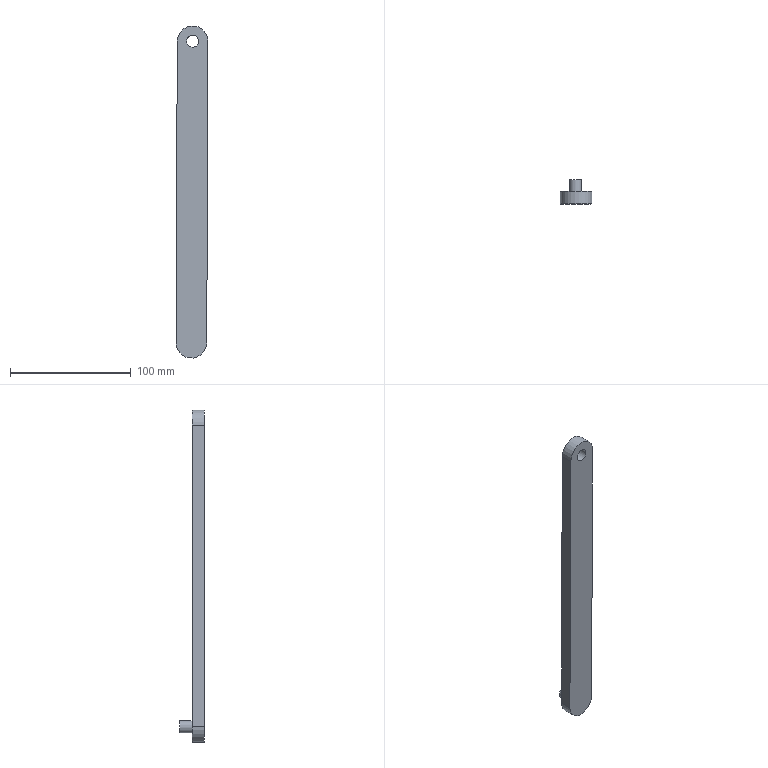Component | NX | 07 | 1 solid | 9 faces | box 26.54 x 20 x 275.49 mm | volume 68832 mm3 | plane 5 | cylinder 4 | commonest cylinder face diameters 25.491 x2 10 x2
STEP:
#1=CARTESIAN_POINT('',(0.,0.,0.));
#2=DIRECTION('',(0.,0.,1.));
#3=DIRECTION('',(1.,0.,0.));
#4=AXIS2_PLACEMENT_3D('',#1,#2,#3);
#5=CARTESIAN_POINT('',(-187.255,5.,90.359));
#6=VERTEX_POINT('',#5);
#7=CARTESIAN_POINT('',(-186.21,5.,340.356));
#8=VERTEX_POINT('',#7);
#9=CARTESIAN_POINT('',(-187.255,5.,90.359));
#10=DIRECTION('',(0.004176,0.,1.));
#11=VECTOR('',#10,1.);
#12=LINE('',#9,#11);
#13=CARTESIAN_POINT('',(-187.255,15.,90.359));
#14=DIRECTION('',(1.,0.,-0.004176));
#15=DIRECTION('',(-0.004176,0.,-1.));
#16=AXIS2_PLACEMENT_3D('',#13,#14,#15);
#17=PLANE('',#16);
#18=CARTESIAN_POINT('',(0.,-10.));
#19=DIRECTION('',(-1.,0.));
#20=VECTOR('',#19,1.);
#21=LINE('',#18,#20);
#22=(GEOMETRIC_REPRESENTATION_CONTEXT(2)PARAMETRIC_REPRESENTATION_CONTEXT()REPRESENTATION_CONTEXT('',''));
#23=DEFINITIONAL_REPRESENTATION('',(#21),#22);
#24=PCURVE('',#17,#23);
#25=CARTESIAN_POINT('',(-198.956,5.,340.41));
#26=DIRECTION('',(0.,-1.,0.));
#27=DIRECTION('',(0.004176,0.,1.));
#28=AXIS2_PLACEMENT_3D('',#25,#26,#27);
#29=PLANE('',#28);
#30=CARTESIAN_POINT('',(-250.,-12.746));
#31=DIRECTION('',(1.,0.));
#32=VECTOR('',#31,1.);
#33=LINE('',#30,#32);
#34=(GEOMETRIC_REPRESENTATION_CONTEXT(2)PARAMETRIC_REPRESENTATION_CONTEXT()REPRESENTATION_CONTEXT('',''));
#35=DEFINITIONAL_REPRESENTATION('',(#33),#34);
#36=PCURVE('',#29,#35);
#37=SURFACE_CURVE('',#12,(#24,#36),.PCURVE_S1.);
#38=EDGE_CURVE('',#6,#8,#37,.T.);
#39=ORIENTED_EDGE('',*,*,#38,.F.);
#40=CARTESIAN_POINT('',(-187.255,15.,90.359));
#41=VERTEX_POINT('',#40);
#42=CARTESIAN_POINT('',(-187.255,15.,90.359));
#43=DIRECTION('',(0.,-1.,0.));
#44=VECTOR('',#43,1.);
#45=LINE('',#42,#44);
#46=CARTESIAN_POINT('',(0.,0.));
#47=DIRECTION('',(0.,-1.));
#48=VECTOR('',#47,1.);
#49=LINE('',#46,#48);
#50=(GEOMETRIC_REPRESENTATION_CONTEXT(2)PARAMETRIC_REPRESENTATION_CONTEXT()REPRESENTATION_CONTEXT('',''));
#51=DEFINITIONAL_REPRESENTATION('',(#49),#50);
#52=PCURVE('',#17,#51);
#53=CARTESIAN_POINT('',(-200.,15.,90.412));
#54=DIRECTION('',(0.,-1.,0.));
#55=DIRECTION('',(0.004176,0.,1.));
#56=AXIS2_PLACEMENT_3D('',#53,#54,#55);
#57=CYLINDRICAL_SURFACE('',#56,12.746);
#58=CARTESIAN_POINT('',(4.712,0.));
#59=DIRECTION('',(0.,1.));
#60=VECTOR('',#59,1.);
#61=LINE('',#58,#60);
#62=(GEOMETRIC_REPRESENTATION_CONTEXT(2)PARAMETRIC_REPRESENTATION_CONTEXT()REPRESENTATION_CONTEXT('',''));
#63=DEFINITIONAL_REPRESENTATION('',(#61),#62);
#64=PCURVE('',#57,#63);
#65=SURFACE_CURVE('',#45,(#52,#64),.PCURVE_S1.);
#66=EDGE_CURVE('',#41,#6,#65,.T.);
#67=ORIENTED_EDGE('',*,*,#66,.F.);
#68=CARTESIAN_POINT('',(-186.21,15.,340.356));
#69=VERTEX_POINT('',#68);
#70=CARTESIAN_POINT('',(-187.255,15.,90.359));
#71=DIRECTION('',(0.004176,0.,1.));
#72=VECTOR('',#71,1.);
#73=LINE('',#70,#72);
#74=CARTESIAN_POINT('',(0.,0.));
#75=DIRECTION('',(-1.,0.));
#76=VECTOR('',#75,1.);
#77=LINE('',#74,#76);
#78=(GEOMETRIC_REPRESENTATION_CONTEXT(2)PARAMETRIC_REPRESENTATION_CONTEXT()REPRESENTATION_CONTEXT('',''));
#79=DEFINITIONAL_REPRESENTATION('',(#77),#78);
#80=PCURVE('',#17,#79);
#81=CARTESIAN_POINT('',(-198.956,15.,340.41));
#82=DIRECTION('',(0.,-1.,0.));
#83=DIRECTION('',(0.004176,0.,1.));
#84=AXIS2_PLACEMENT_3D('',#81,#82,#83);
#85=PLANE('',#84);
#86=CARTESIAN_POINT('',(-250.,-12.746));
#87=DIRECTION('',(1.,0.));
#88=VECTOR('',#87,1.);
#89=LINE('',#86,#88);
#90=(GEOMETRIC_REPRESENTATION_CONTEXT(2)PARAMETRIC_REPRESENTATION_CONTEXT()REPRESENTATION_CONTEXT('',''));
#91=DEFINITIONAL_REPRESENTATION('',(#89),#90);
#92=PCURVE('',#85,#91);
#93=SURFACE_CURVE('',#73,(#80,#92),.PCURVE_S1.);
#94=EDGE_CURVE('',#41,#69,#93,.T.);
#95=ORIENTED_EDGE('',*,*,#94,.T.);
#96=CARTESIAN_POINT('',(-186.21,15.,340.356));
#97=DIRECTION('',(0.,-1.,0.));
#98=VECTOR('',#97,1.);
#99=LINE('',#96,#98);
#100=CARTESIAN_POINT('',(-250.,0.));
#101=DIRECTION('',(0.,-1.));
#102=VECTOR('',#101,1.);
#103=LINE('',#100,#102);
#104=(GEOMETRIC_REPRESENTATION_CONTEXT(2)PARAMETRIC_REPRESENTATION_CONTEXT()REPRESENTATION_CONTEXT('',''));
#105=DEFINITIONAL_REPRESENTATION('',(#103),#104);
#106=PCURVE('',#17,#105);
#107=CARTESIAN_POINT('',(-198.956,15.,340.41));
#108=DIRECTION('',(0.,-1.,0.));
#109=DIRECTION('',(0.004176,0.,1.));
#110=AXIS2_PLACEMENT_3D('',#107,#108,#109);
#111=CYLINDRICAL_SURFACE('',#110,12.746);
#112=CARTESIAN_POINT('',(-1.571,0.));
#113=DIRECTION('',(0.,1.));
#114=VECTOR('',#113,1.);
#115=LINE('',#112,#114);
#116=(GEOMETRIC_REPRESENTATION_CONTEXT(2)PARAMETRIC_REPRESENTATION_CONTEXT()REPRESENTATION_CONTEXT('',''));
#117=DEFINITIONAL_REPRESENTATION('',(#115),#116);
#118=PCURVE('',#111,#117);
#119=SURFACE_CURVE('',#99,(#106,#118),.PCURVE_S1.);
#120=EDGE_CURVE('',#69,#8,#119,.T.);
#121=ORIENTED_EDGE('',*,*,#120,.T.);
#122=EDGE_LOOP('',(#39,#67,#95,#121));
#123=FACE_BOUND('',#122,.T.);
#124=ADVANCED_FACE('',(#123),#17,.T.);
#125=CARTESIAN_POINT('',(-211.701,5.,340.463));
#126=VERTEX_POINT('',#125);
#127=CARTESIAN_POINT('',(-198.956,5.,340.41));
#128=DIRECTION('',(0.,-1.,0.));
#129=DIRECTION('',(-1.,0.,0.004176));
#130=AXIS2_PLACEMENT_3D('',#127,#128,#129);
#131=CIRCLE('',#130,12.746);
#132=CARTESIAN_POINT('',(-4.712,10.));
#133=DIRECTION('',(1.,0.));
#134=VECTOR('',#133,1.);
#135=LINE('',#132,#134);
#136=(GEOMETRIC_REPRESENTATION_CONTEXT(2)PARAMETRIC_REPRESENTATION_CONTEXT()REPRESENTATION_CONTEXT('',''));
#137=DEFINITIONAL_REPRESENTATION('',(#135),#136);
#138=PCURVE('',#111,#137);
#139=CARTESIAN_POINT('',(0.,0.));
#140=DIRECTION('',(0.,1.));
#141=AXIS2_PLACEMENT_2D('',#139,#140);
#142=CIRCLE('',#141,12.746);
#143=(GEOMETRIC_REPRESENTATION_CONTEXT(2)PARAMETRIC_REPRESENTATION_CONTEXT()REPRESENTATION_CONTEXT('',''));
#144=DEFINITIONAL_REPRESENTATION('',(#142),#143);
#145=PCURVE('',#29,#144);
#146=SURFACE_CURVE('',#131,(#138,#145),.PCURVE_S1.);
#147=EDGE_CURVE('',#8,#126,#146,.T.);
#148=ORIENTED_EDGE('',*,*,#147,.F.);
#149=ORIENTED_EDGE('',*,*,#120,.F.);
#150=CARTESIAN_POINT('',(-211.701,15.,340.463));
#151=VERTEX_POINT('',#150);
#152=CARTESIAN_POINT('',(-198.956,15.,340.41));
#153=DIRECTION('',(0.,-1.,0.));
#154=DIRECTION('',(-1.,0.,0.004176));
#155=AXIS2_PLACEMENT_3D('',#152,#153,#154);
#156=CIRCLE('',#155,12.746);
#157=CARTESIAN_POINT('',(-4.712,0.));
#158=DIRECTION('',(1.,0.));
#159=VECTOR('',#158,1.);
#160=LINE('',#157,#159);
#161=(GEOMETRIC_REPRESENTATION_CONTEXT(2)PARAMETRIC_REPRESENTATION_CONTEXT()REPRESENTATION_CONTEXT('',''));
#162=DEFINITIONAL_REPRESENTATION('',(#160),#161);
#163=PCURVE('',#111,#162);
#164=CARTESIAN_POINT('',(0.,0.));
#165=DIRECTION('',(0.,1.));
#166=AXIS2_PLACEMENT_2D('',#164,#165);
#167=CIRCLE('',#166,12.746);
#168=(GEOMETRIC_REPRESENTATION_CONTEXT(2)PARAMETRIC_REPRESENTATION_CONTEXT()REPRESENTATION_CONTEXT('',''));
#169=DEFINITIONAL_REPRESENTATION('',(#167),#168);
#170=PCURVE('',#85,#169);
#171=SURFACE_CURVE('',#156,(#163,#170),.PCURVE_S1.);
#172=EDGE_CURVE('',#69,#151,#171,.T.);
#173=ORIENTED_EDGE('',*,*,#172,.T.);
#174=CARTESIAN_POINT('',(-211.701,15.,340.463));
#175=DIRECTION('',(0.,-1.,0.));
#176=VECTOR('',#175,1.);
#177=LINE('',#174,#176);
#178=CARTESIAN_POINT('',(1.571,0.));
#179=DIRECTION('',(0.,1.));
#180=VECTOR('',#179,1.);
#181=LINE('',#178,#180);
#182=(GEOMETRIC_REPRESENTATION_CONTEXT(2)PARAMETRIC_REPRESENTATION_CONTEXT()REPRESENTATION_CONTEXT('',''));
#183=DEFINITIONAL_REPRESENTATION('',(#181),#182);
#184=PCURVE('',#111,#183);
#185=CARTESIAN_POINT('',(-211.701,15.,340.463));
#186=DIRECTION('',(-1.,0.,0.004176));
#187=DIRECTION('',(0.004176,0.,1.));
#188=AXIS2_PLACEMENT_3D('',#185,#186,#187);
#189=PLANE('',#188);
#190=CARTESIAN_POINT('',(0.,0.));
#191=DIRECTION('',(0.,-1.));
#192=VECTOR('',#191,1.);
#193=LINE('',#190,#192);
#194=(GEOMETRIC_REPRESENTATION_CONTEXT(2)PARAMETRIC_REPRESENTATION_CONTEXT()REPRESENTATION_CONTEXT('',''));
#195=DEFINITIONAL_REPRESENTATION('',(#193),#194);
#196=PCURVE('',#189,#195);
#197=SURFACE_CURVE('',#177,(#184,#196),.PCURVE_S1.);
#198=EDGE_CURVE('',#151,#126,#197,.T.);
#199=ORIENTED_EDGE('',*,*,#198,.T.);
#200=EDGE_LOOP('',(#148,#149,#173,#199));
#201=FACE_BOUND('',#200,.T.);
#202=ADVANCED_FACE('',(#201),#111,.T.);
#203=CARTESIAN_POINT('',(-212.745,5.,90.465));
#204=VERTEX_POINT('',#203);
#205=CARTESIAN_POINT('',(-211.701,5.,340.463));
#206=DIRECTION('',(-0.004176,0.,-1.));
#207=VECTOR('',#206,1.);
#208=LINE('',#205,#207);
#209=CARTESIAN_POINT('',(0.,-10.));
#210=DIRECTION('',(-1.,0.));
#211=VECTOR('',#210,1.);
#212=LINE('',#209,#211);
#213=(GEOMETRIC_REPRESENTATION_CONTEXT(2)PARAMETRIC_REPRESENTATION_CONTEXT()REPRESENTATION_CONTEXT('',''));
#214=DEFINITIONAL_REPRESENTATION('',(#212),#213);
#215=PCURVE('',#189,#214);
#216=CARTESIAN_POINT('',(-0.,12.746));
#217=DIRECTION('',(-1.,-0.));
#218=VECTOR('',#217,1.);
#219=LINE('',#216,#218);
#220=(GEOMETRIC_REPRESENTATION_CONTEXT(2)PARAMETRIC_REPRESENTATION_CONTEXT()REPRESENTATION_CONTEXT('',''));
#221=DEFINITIONAL_REPRESENTATION('',(#219),#220);
#222=PCURVE('',#29,#221);
#223=SURFACE_CURVE('',#208,(#215,#222),.PCURVE_S1.);
#224=EDGE_CURVE('',#126,#204,#223,.T.);
#225=ORIENTED_EDGE('',*,*,#224,.F.);
#226=ORIENTED_EDGE('',*,*,#198,.F.);
#227=CARTESIAN_POINT('',(-212.745,15.,90.465));
#228=VERTEX_POINT('',#227);
#229=CARTESIAN_POINT('',(-211.701,15.,340.463));
#230=DIRECTION('',(-0.004176,0.,-1.));
#231=VECTOR('',#230,1.);
#232=LINE('',#229,#231);
#233=CARTESIAN_POINT('',(0.,0.));
#234=DIRECTION('',(-1.,0.));
#235=VECTOR('',#234,1.);
#236=LINE('',#233,#235);
#237=(GEOMETRIC_REPRESENTATION_CONTEXT(2)PARAMETRIC_REPRESENTATION_CONTEXT()REPRESENTATION_CONTEXT('',''));
#238=DEFINITIONAL_REPRESENTATION('',(#236),#237);
#239=PCURVE('',#189,#238);
#240=CARTESIAN_POINT('',(-0.,12.746));
#241=DIRECTION('',(-1.,-0.));
#242=VECTOR('',#241,1.);
#243=LINE('',#240,#242);
#244=(GEOMETRIC_REPRESENTATION_CONTEXT(2)PARAMETRIC_REPRESENTATION_CONTEXT()REPRESENTATION_CONTEXT('',''));
#245=DEFINITIONAL_REPRESENTATION('',(#243),#244);
#246=PCURVE('',#85,#245);
#247=SURFACE_CURVE('',#232,(#239,#246),.PCURVE_S1.);
#248=EDGE_CURVE('',#151,#228,#247,.T.);
#249=ORIENTED_EDGE('',*,*,#248,.T.);
#250=CARTESIAN_POINT('',(-212.745,15.,90.465));
#251=DIRECTION('',(0.,-1.,0.));
#252=VECTOR('',#251,1.);
#253=LINE('',#250,#252);
#254=CARTESIAN_POINT('',(-250.,0.));
#255=DIRECTION('',(0.,-1.));
#256=VECTOR('',#255,1.);
#257=LINE('',#254,#256);
#258=(GEOMETRIC_REPRESENTATION_CONTEXT(2)PARAMETRIC_REPRESENTATION_CONTEXT()REPRESENTATION_CONTEXT('',''));
#259=DEFINITIONAL_REPRESENTATION('',(#257),#258);
#260=PCURVE('',#189,#259);
#261=CARTESIAN_POINT('',(1.571,0.));
#262=DIRECTION('',(0.,1.));
#263=VECTOR('',#262,1.);
#264=LINE('',#261,#263);
#265=(GEOMETRIC_REPRESENTATION_CONTEXT(2)PARAMETRIC_REPRESENTATION_CONTEXT()REPRESENTATION_CONTEXT('',''));
#266=DEFINITIONAL_REPRESENTATION('',(#264),#265);
#267=PCURVE('',#57,#266);
#268=SURFACE_CURVE('',#253,(#260,#267),.PCURVE_S1.);
#269=EDGE_CURVE('',#228,#204,#268,.T.);
#270=ORIENTED_EDGE('',*,*,#269,.T.);
#271=EDGE_LOOP('',(#225,#226,#249,#270));
#272=FACE_BOUND('',#271,.T.);
#273=ADVANCED_FACE('',(#272),#189,.T.);
#274=CARTESIAN_POINT('',(-200.,5.,90.412));
#275=DIRECTION('',(0.,-1.,0.));
#276=DIRECTION('',(-1.,0.,0.004176));
#277=AXIS2_PLACEMENT_3D('',#274,#275,#276);
#278=CIRCLE('',#277,12.746);
#279=CARTESIAN_POINT('',(1.571,10.));
#280=DIRECTION('',(1.,0.));
#281=VECTOR('',#280,1.);
#282=LINE('',#279,#281);
#283=(GEOMETRIC_REPRESENTATION_CONTEXT(2)PARAMETRIC_REPRESENTATION_CONTEXT()REPRESENTATION_CONTEXT('',''));
#284=DEFINITIONAL_REPRESENTATION('',(#282),#283);
#285=PCURVE('',#57,#284);
#286=CARTESIAN_POINT('',(-250.,0.));
#287=DIRECTION('',(0.,1.));
#288=AXIS2_PLACEMENT_2D('',#286,#287);
#289=CIRCLE('',#288,12.746);
#290=(GEOMETRIC_REPRESENTATION_CONTEXT(2)PARAMETRIC_REPRESENTATION_CONTEXT()REPRESENTATION_CONTEXT('',''));
#291=DEFINITIONAL_REPRESENTATION('',(#289),#290);
#292=PCURVE('',#29,#291);
#293=SURFACE_CURVE('',#278,(#285,#292),.PCURVE_S1.);
#294=EDGE_CURVE('',#204,#6,#293,.T.);
#295=ORIENTED_EDGE('',*,*,#294,.F.);
#296=ORIENTED_EDGE('',*,*,#269,.F.);
#297=CARTESIAN_POINT('',(-200.,15.,90.412));
#298=DIRECTION('',(0.,-1.,0.));
#299=DIRECTION('',(-1.,0.,0.004176));
#300=AXIS2_PLACEMENT_3D('',#297,#298,#299);
#301=CIRCLE('',#300,12.746);
#302=CARTESIAN_POINT('',(1.571,0.));
#303=DIRECTION('',(1.,0.));
#304=VECTOR('',#303,1.);
#305=LINE('',#302,#304);
#306=(GEOMETRIC_REPRESENTATION_CONTEXT(2)PARAMETRIC_REPRESENTATION_CONTEXT()REPRESENTATION_CONTEXT('',''));
#307=DEFINITIONAL_REPRESENTATION('',(#305),#306);
#308=PCURVE('',#57,#307);
#309=CARTESIAN_POINT('',(-250.,0.));
#310=DIRECTION('',(0.,1.));
#311=AXIS2_PLACEMENT_2D('',#309,#310);
#312=CIRCLE('',#311,12.746);
#313=(GEOMETRIC_REPRESENTATION_CONTEXT(2)PARAMETRIC_REPRESENTATION_CONTEXT()REPRESENTATION_CONTEXT('',''));
#314=DEFINITIONAL_REPRESENTATION('',(#312),#313);
#315=PCURVE('',#85,#314);
#316=SURFACE_CURVE('',#301,(#308,#315),.PCURVE_S1.);
#317=EDGE_CURVE('',#228,#41,#316,.T.);
#318=ORIENTED_EDGE('',*,*,#317,.T.);
#319=ORIENTED_EDGE('',*,*,#66,.T.);
#320=EDGE_LOOP('',(#295,#296,#318,#319));
#321=FACE_BOUND('',#320,.T.);
#322=ADVANCED_FACE('',(#321),#57,.T.);
#323=CARTESIAN_POINT('',(-205.,15.,90.433));
#324=VERTEX_POINT('',#323);
#325=CARTESIAN_POINT('',(-200.,15.,90.412));
#326=DIRECTION('',(0.,1.,0.));
#327=DIRECTION('',(-1.,0.,0.004176));
#328=AXIS2_PLACEMENT_3D('',#325,#326,#327);
#329=CIRCLE('',#328,5.);
#330=CARTESIAN_POINT('',(-250.,5.));
#331=CARTESIAN_POINT('',(-241.34,5.));
#332=CARTESIAN_POINT('',(-245.67,-2.5));
#333=CARTESIAN_POINT('',(-250.,-10.));
#334=CARTESIAN_POINT('',(-254.33,-2.5));
#335=CARTESIAN_POINT('',(-258.66,5.));
#336=CARTESIAN_POINT('',(-250.,5.));
#337=(BOUNDED_CURVE()B_SPLINE_CURVE(2,(#330,#331,#332,#333,#334,#335,#336),.UNSPECIFIED.,.T.,.F.)B_SPLINE_CURVE_WITH_KNOTS((1,2,2,2,2,1),(-2.094,0.,2.094,4.189,6.283,8.378),.UNSPECIFIED.)CURVE()GEOMETRIC_REPRESENTATION_ITEM()RATIONAL_B_SPLINE_CURVE((1.,0.5,1.,0.5,1.,0.5,1.))REPRESENTATION_ITEM(''));
#338=(GEOMETRIC_REPRESENTATION_CONTEXT(2)PARAMETRIC_REPRESENTATION_CONTEXT()REPRESENTATION_CONTEXT('',''));
#339=DEFINITIONAL_REPRESENTATION('',(#337),#338);
#340=PCURVE('',#85,#339);
#341=CARTESIAN_POINT('',(-200.,25.,90.412));
#342=DIRECTION('',(0.,-1.,0.));
#343=DIRECTION('',(0.004176,0.,1.));
#344=AXIS2_PLACEMENT_3D('',#341,#342,#343);
#345=CYLINDRICAL_SURFACE('',#344,5.);
#346=CARTESIAN_POINT('',(7.854,10.));
#347=DIRECTION('',(-1.,0.));
#348=VECTOR('',#347,1.);
#349=LINE('',#346,#348);
#350=(GEOMETRIC_REPRESENTATION_CONTEXT(2)PARAMETRIC_REPRESENTATION_CONTEXT()REPRESENTATION_CONTEXT('',''));
#351=DEFINITIONAL_REPRESENTATION('',(#349),#350);
#352=PCURVE('',#345,#351);
#353=SURFACE_CURVE('',#329,(#340,#352),.PCURVE_S1.);
#354=EDGE_CURVE('',#324,#324,#353,.T.);
#355=ORIENTED_EDGE('',*,*,#354,.F.);
#356=EDGE_LOOP('',(#355));
#357=FACE_BOUND('',#356,.T.);
#358=CARTESIAN_POINT('',(-203.956,15.,340.431));
#359=VERTEX_POINT('',#358);
#360=CARTESIAN_POINT('',(-198.956,15.,340.41));
#361=DIRECTION('',(0.,1.,0.));
#362=DIRECTION('',(-1.,0.,0.004176));
#363=AXIS2_PLACEMENT_3D('',#360,#361,#362);
#364=CIRCLE('',#363,5.);
#365=CARTESIAN_POINT('',(0.,5.));
#366=CARTESIAN_POINT('',(8.66,5.));
#367=CARTESIAN_POINT('',(4.33,-2.5));
#368=CARTESIAN_POINT('',(-0.,-10.));
#369=CARTESIAN_POINT('',(-4.33,-2.5));
#370=CARTESIAN_POINT('',(-8.66,5.));
#371=CARTESIAN_POINT('',(0.,5.));
#372=(BOUNDED_CURVE()B_SPLINE_CURVE(2,(#365,#366,#367,#368,#369,#370,#371),.UNSPECIFIED.,.T.,.F.)B_SPLINE_CURVE_WITH_KNOTS((1,2,2,2,2,1),(-2.094,0.,2.094,4.189,6.283,8.378),.UNSPECIFIED.)CURVE()GEOMETRIC_REPRESENTATION_ITEM()RATIONAL_B_SPLINE_CURVE((1.,0.5,1.,0.5,1.,0.5,1.))REPRESENTATION_ITEM(''));
#373=(GEOMETRIC_REPRESENTATION_CONTEXT(2)PARAMETRIC_REPRESENTATION_CONTEXT()REPRESENTATION_CONTEXT('',''));
#374=DEFINITIONAL_REPRESENTATION('',(#372),#373);
#375=PCURVE('',#85,#374);
#376=CARTESIAN_POINT('',(-198.956,-84.,340.41));
#377=DIRECTION('',(0.,1.,0.));
#378=DIRECTION('',(-0.004176,0.,-1.));
#379=AXIS2_PLACEMENT_3D('',#376,#377,#378);
#380=CYLINDRICAL_SURFACE('',#379,5.);
#381=CARTESIAN_POINT('',(1.571,99.));
#382=DIRECTION('',(1.,0.));
#383=VECTOR('',#382,1.);
#384=LINE('',#381,#383);
#385=(GEOMETRIC_REPRESENTATION_CONTEXT(2)PARAMETRIC_REPRESENTATION_CONTEXT()REPRESENTATION_CONTEXT('',''));
#386=DEFINITIONAL_REPRESENTATION('',(#384),#385);
#387=PCURVE('',#380,#386);
#388=SURFACE_CURVE('',#364,(#375,#387),.PCURVE_S1.);
#389=EDGE_CURVE('',#359,#359,#388,.T.);
#390=ORIENTED_EDGE('',*,*,#389,.F.);
#391=EDGE_LOOP('',(#390));
#392=FACE_BOUND('',#391,.T.);
#393=ORIENTED_EDGE('',*,*,#94,.F.);
#394=ORIENTED_EDGE('',*,*,#317,.F.);
#395=ORIENTED_EDGE('',*,*,#248,.F.);
#396=ORIENTED_EDGE('',*,*,#172,.F.);
#397=EDGE_LOOP('',(#393,#394,#395,#396));
#398=FACE_BOUND('',#397,.T.);
#399=ADVANCED_FACE('',(#357,#392,#398),#85,.F.);
#400=CARTESIAN_POINT('',(-198.935,5.,345.41));
#401=VERTEX_POINT('',#400);
#402=CARTESIAN_POINT('',(-203.956,5.,340.431));
#403=VERTEX_POINT('',#402);
#404=CARTESIAN_POINT('',(-198.956,5.,340.41));
#405=DIRECTION('',(0.,1.,0.));
#406=DIRECTION('',(0.004176,0.,1.));
#407=AXIS2_PLACEMENT_3D('',#404,#405,#406);
#408=CIRCLE('',#407,5.);
#409=CARTESIAN_POINT('',(5.,0.));
#410=CARTESIAN_POINT('',(5.,-8.66));
#411=CARTESIAN_POINT('',(-2.5,-4.33));
#412=CARTESIAN_POINT('',(-10.,-0.));
#413=CARTESIAN_POINT('',(-2.5,4.33));
#414=CARTESIAN_POINT('',(5.,8.66));
#415=CARTESIAN_POINT('',(5.,0.));
#416=(BOUNDED_CURVE()B_SPLINE_CURVE(2,(#409,#410,#411,#412,#413,#414,#415),.UNSPECIFIED.,.T.,.F.)B_SPLINE_CURVE_WITH_KNOTS((1,2,2,2,2,1),(-2.094,0.,2.094,4.189,6.283,8.378),.UNSPECIFIED.)CURVE()GEOMETRIC_REPRESENTATION_ITEM()RATIONAL_B_SPLINE_CURVE((1.,0.5,1.,0.5,1.,0.5,1.))REPRESENTATION_ITEM(''));
#417=(GEOMETRIC_REPRESENTATION_CONTEXT(2)PARAMETRIC_REPRESENTATION_CONTEXT()REPRESENTATION_CONTEXT('',''));
#418=DEFINITIONAL_REPRESENTATION('',(#416),#417);
#419=PCURVE('',#29,#418);
#420=CARTESIAN_POINT('',(3.142,89.));
#421=DIRECTION('',(1.,0.));
#422=VECTOR('',#421,1.);
#423=LINE('',#420,#422);
#424=(GEOMETRIC_REPRESENTATION_CONTEXT(2)PARAMETRIC_REPRESENTATION_CONTEXT()REPRESENTATION_CONTEXT('',''));
#425=DEFINITIONAL_REPRESENTATION('',(#423),#424);
#426=PCURVE('',#380,#425);
#427=SURFACE_CURVE('',#408,(#419,#426),.PCURVE_S1.);
#428=EDGE_CURVE('',#401,#403,#427,.T.);
#429=ORIENTED_EDGE('',*,*,#428,.T.);
#430=CARTESIAN_POINT('',(-198.956,5.,340.41));
#431=DIRECTION('',(0.,1.,0.));
#432=DIRECTION('',(0.004176,0.,1.));
#433=AXIS2_PLACEMENT_3D('',#430,#431,#432);
#434=CIRCLE('',#433,5.);
#435=CARTESIAN_POINT('',(5.,0.));
#436=CARTESIAN_POINT('',(5.,-8.66));
#437=CARTESIAN_POINT('',(-2.5,-4.33));
#438=CARTESIAN_POINT('',(-10.,-0.));
#439=CARTESIAN_POINT('',(-2.5,4.33));
#440=CARTESIAN_POINT('',(5.,8.66));
#441=CARTESIAN_POINT('',(5.,0.));
#442=(BOUNDED_CURVE()B_SPLINE_CURVE(2,(#435,#436,#437,#438,#439,#440,#441),.UNSPECIFIED.,.T.,.F.)B_SPLINE_CURVE_WITH_KNOTS((1,2,2,2,2,1),(-2.094,0.,2.094,4.189,6.283,8.378),.UNSPECIFIED.)CURVE()GEOMETRIC_REPRESENTATION_ITEM()RATIONAL_B_SPLINE_CURVE((1.,0.5,1.,0.5,1.,0.5,1.))REPRESENTATION_ITEM(''));
#443=(GEOMETRIC_REPRESENTATION_CONTEXT(2)PARAMETRIC_REPRESENTATION_CONTEXT()REPRESENTATION_CONTEXT('',''));
#444=DEFINITIONAL_REPRESENTATION('',(#442),#443);
#445=PCURVE('',#29,#444);
#446=CARTESIAN_POINT('',(-3.142,89.));
#447=DIRECTION('',(1.,0.));
#448=VECTOR('',#447,1.);
#449=LINE('',#446,#448);
#450=(GEOMETRIC_REPRESENTATION_CONTEXT(2)PARAMETRIC_REPRESENTATION_CONTEXT()REPRESENTATION_CONTEXT('',''));
#451=DEFINITIONAL_REPRESENTATION('',(#449),#450);
#452=PCURVE('',#380,#451);
#453=SURFACE_CURVE('',#434,(#445,#452),.PCURVE_S1.);
#454=EDGE_CURVE('',#403,#401,#453,.T.);
#455=ORIENTED_EDGE('',*,*,#454,.T.);
#456=EDGE_LOOP('',(#429,#455));
#457=FACE_BOUND('',#456,.T.);
#458=ORIENTED_EDGE('',*,*,#38,.T.);
#459=ORIENTED_EDGE('',*,*,#147,.T.);
#460=ORIENTED_EDGE('',*,*,#224,.T.);
#461=ORIENTED_EDGE('',*,*,#294,.T.);
#462=EDGE_LOOP('',(#458,#459,#460,#461));
#463=FACE_BOUND('',#462,.T.);
#464=ADVANCED_FACE('',(#457,#463),#29,.T.);
#465=ORIENTED_EDGE('',*,*,#389,.F.);
#466=CARTESIAN_POINT('',(-203.956,5.,340.431));
#467=CARTESIAN_POINT('',(-203.956,15.,340.431));
#468=B_SPLINE_CURVE_WITH_KNOTS('',1,(#466,#467),.UNSPECIFIED.,.F.,.F.,(2,2),(89.,99.),.PIECEWISE_BEZIER_KNOTS.);
#469=CARTESIAN_POINT('',(1.571,0.));
#470=DIRECTION('',(0.,1.));
#471=VECTOR('',#470,1.);
#472=LINE('',#469,#471);
#473=(GEOMETRIC_REPRESENTATION_CONTEXT(2)PARAMETRIC_REPRESENTATION_CONTEXT()REPRESENTATION_CONTEXT('',''));
#474=DEFINITIONAL_REPRESENTATION('',(#472),#473);
#475=PCURVE('',#380,#474);
#476=CARTESIAN_POINT('',(7.854,0.));
#477=DIRECTION('',(0.,1.));
#478=VECTOR('',#477,1.);
#479=LINE('',#476,#478);
#480=(GEOMETRIC_REPRESENTATION_CONTEXT(2)PARAMETRIC_REPRESENTATION_CONTEXT()REPRESENTATION_CONTEXT('',''));
#481=DEFINITIONAL_REPRESENTATION('',(#479),#480);
#482=PCURVE('',#380,#481);
#483=SEAM_CURVE('',#468,(#475,#482),.PCURVE_S1.);
#484=EDGE_CURVE('',#403,#359,#483,.T.);
#485=ORIENTED_EDGE('',*,*,#484,.F.);
#486=ORIENTED_EDGE('',*,*,#454,.T.);
#487=ORIENTED_EDGE('',*,*,#428,.T.);
#488=ORIENTED_EDGE('',*,*,#484,.T.);
#489=EDGE_LOOP('',(#465,#485,#486,#487,#488));
#490=FACE_BOUND('',#489,.F.);
#491=ADVANCED_FACE('',(#490),#380,.F.);
#492=CARTESIAN_POINT('',(-205.,25.,90.433));
#493=VERTEX_POINT('',#492);
#494=CARTESIAN_POINT('',(-200.,25.,90.412));
#495=DIRECTION('',(0.,1.,0.));
#496=DIRECTION('',(-1.,0.,0.004176));
#497=AXIS2_PLACEMENT_3D('',#494,#495,#496);
#498=CIRCLE('',#497,5.);
#499=CARTESIAN_POINT('',(7.854,0.));
#500=DIRECTION('',(-1.,0.));
#501=VECTOR('',#500,1.);
#502=LINE('',#499,#501);
#503=(GEOMETRIC_REPRESENTATION_CONTEXT(2)PARAMETRIC_REPRESENTATION_CONTEXT()REPRESENTATION_CONTEXT('',''));
#504=DEFINITIONAL_REPRESENTATION('',(#502),#503);
#505=PCURVE('',#345,#504);
#506=CARTESIAN_POINT('',(-200.,25.,90.412));
#507=DIRECTION('',(0.,1.,0.));
#508=DIRECTION('',(-0.004176,0.,-1.));
#509=AXIS2_PLACEMENT_3D('',#506,#507,#508);
#510=PLANE('',#509);
#511=CARTESIAN_POINT('',(0.,0.));
#512=DIRECTION('',(-0.,1.));
#513=AXIS2_PLACEMENT_2D('',#511,#512);
#514=CIRCLE('',#513,5.);
#515=(GEOMETRIC_REPRESENTATION_CONTEXT(2)PARAMETRIC_REPRESENTATION_CONTEXT()REPRESENTATION_CONTEXT('',''));
#516=DEFINITIONAL_REPRESENTATION('',(#514),#515);
#517=PCURVE('',#510,#516);
#518=SURFACE_CURVE('',#498,(#505,#517),.PCURVE_S1.);
#519=EDGE_CURVE('',#493,#493,#518,.T.);
#520=ORIENTED_EDGE('',*,*,#519,.F.);
#521=CARTESIAN_POINT('',(-205.,25.,90.433));
#522=CARTESIAN_POINT('',(-205.,15.,90.433));
#523=B_SPLINE_CURVE_WITH_KNOTS('',1,(#521,#522),.UNSPECIFIED.,.F.,.F.,(2,2),(0.,10.),.PIECEWISE_BEZIER_KNOTS.);
#524=CARTESIAN_POINT('',(7.854,0.));
#525=DIRECTION('',(0.,1.));
#526=VECTOR('',#525,1.);
#527=LINE('',#524,#526);
#528=(GEOMETRIC_REPRESENTATION_CONTEXT(2)PARAMETRIC_REPRESENTATION_CONTEXT()REPRESENTATION_CONTEXT('',''));
#529=DEFINITIONAL_REPRESENTATION('',(#527),#528);
#530=PCURVE('',#345,#529);
#531=CARTESIAN_POINT('',(1.571,0.));
#532=DIRECTION('',(0.,1.));
#533=VECTOR('',#532,1.);
#534=LINE('',#531,#533);
#535=(GEOMETRIC_REPRESENTATION_CONTEXT(2)PARAMETRIC_REPRESENTATION_CONTEXT()REPRESENTATION_CONTEXT('',''));
#536=DEFINITIONAL_REPRESENTATION('',(#534),#535);
#537=PCURVE('',#345,#536);
#538=SEAM_CURVE('',#523,(#530,#537),.PCURVE_S1.);
#539=EDGE_CURVE('',#493,#324,#538,.T.);
#540=ORIENTED_EDGE('',*,*,#539,.T.);
#541=ORIENTED_EDGE('',*,*,#354,.T.);
#542=ORIENTED_EDGE('',*,*,#539,.F.);
#543=EDGE_LOOP('',(#520,#540,#541,#542));
#544=FACE_BOUND('',#543,.T.);
#545=ADVANCED_FACE('',(#544),#345,.T.);
#546=ORIENTED_EDGE('',*,*,#519,.T.);
#547=EDGE_LOOP('',(#546));
#548=FACE_BOUND('',#547,.T.);
#549=ADVANCED_FACE('',(#548),#510,.T.);
#550=CLOSED_SHELL('',(#124,#202,#273,#322,#399,#464,#491,#545,#549));
#551=MANIFOLD_SOLID_BREP('',#550);
#552=(LENGTH_UNIT()NAMED_UNIT(*)SI_UNIT(.MILLI.,.METRE.));
#553=UNCERTAINTY_MEASURE_WITH_UNIT(LENGTH_MEASURE(0.000002),#552,'','');
#554=(NAMED_UNIT(*)PLANE_ANGLE_UNIT()SI_UNIT($,.RADIAN.));
#555=(NAMED_UNIT(*)SI_UNIT($,.STERADIAN.)SOLID_ANGLE_UNIT());
#556=(GEOMETRIC_REPRESENTATION_CONTEXT(3)GLOBAL_UNCERTAINTY_ASSIGNED_CONTEXT((#553))GLOBAL_UNIT_ASSIGNED_CONTEXT((#552,#554,#555))REPRESENTATION_CONTEXT('',''));
#557=ADVANCED_BREP_SHAPE_REPRESENTATION('',(#4,#551),#556);